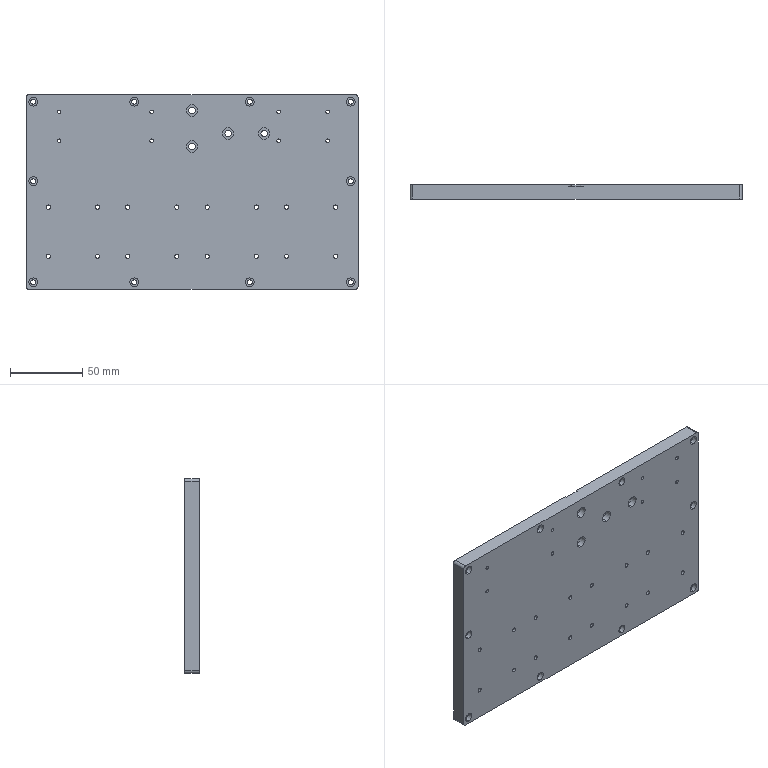CAM job | Mastercam | mm | 15 operations | part box 230 x 10 x 135
1. 2D High Speed (2D Dynamic Contour Mill) | 9 - 10C 平底刀
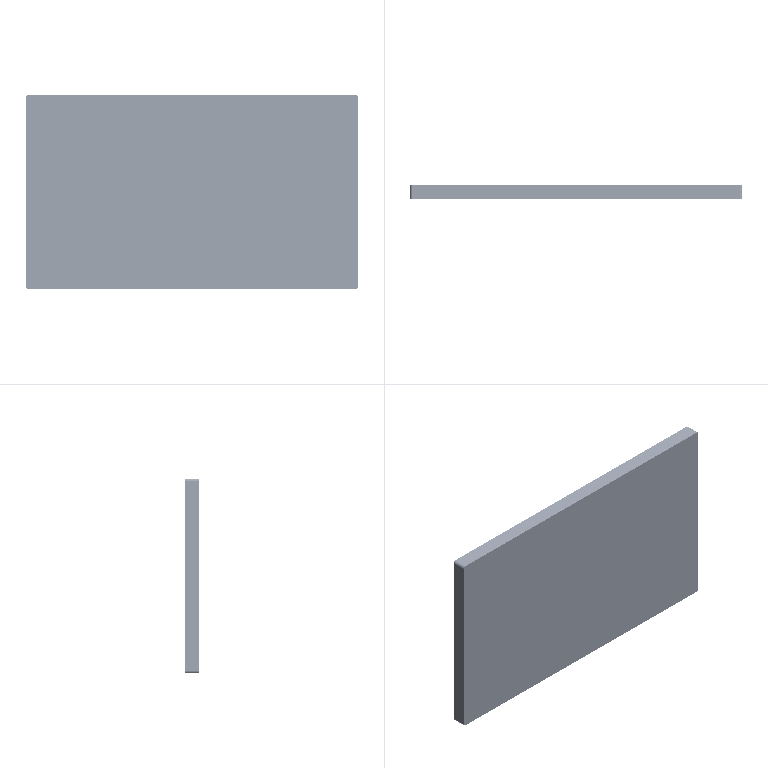2. Contour (2D) | 10 - 10J 平底刀
3. Drill/Counterbore | 2 - 6定位倒角
4. Peck Drill | 12 - 2.5 钻头
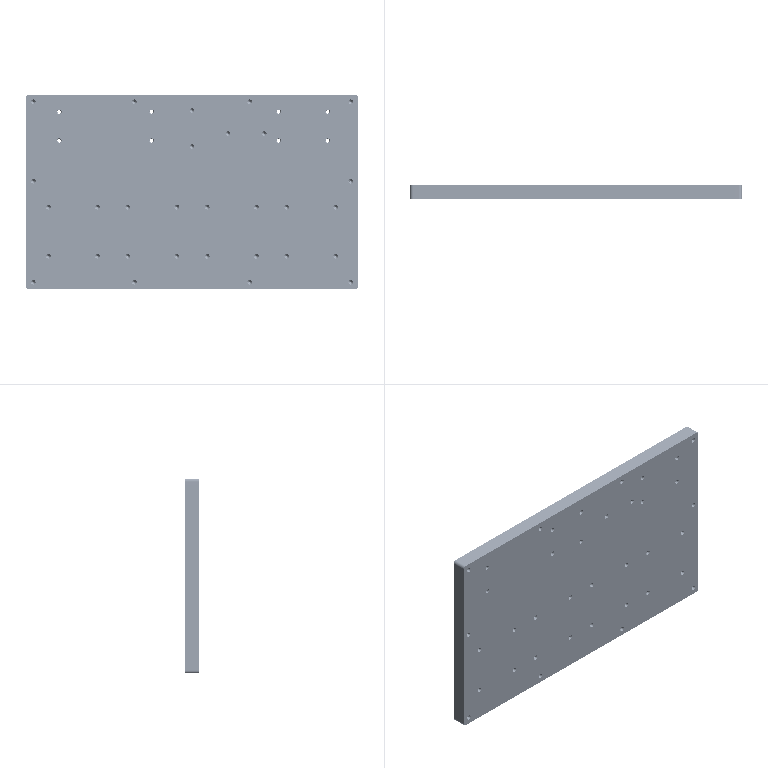5. Peck Drill | 18 - 4.5 钻头
6. Peck Drill | 13 - 3.4 钻头
7. Peck Drill | 19 - 3 钻头
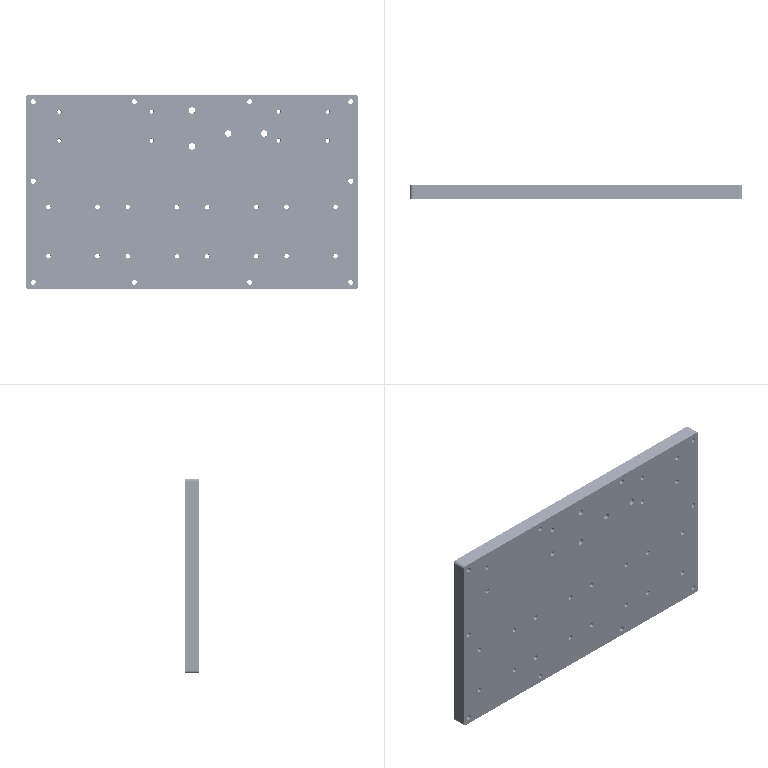8. Helix Bore | 7 - 4 平底刀
9. Model Chamfer | 2 - 6定位倒角
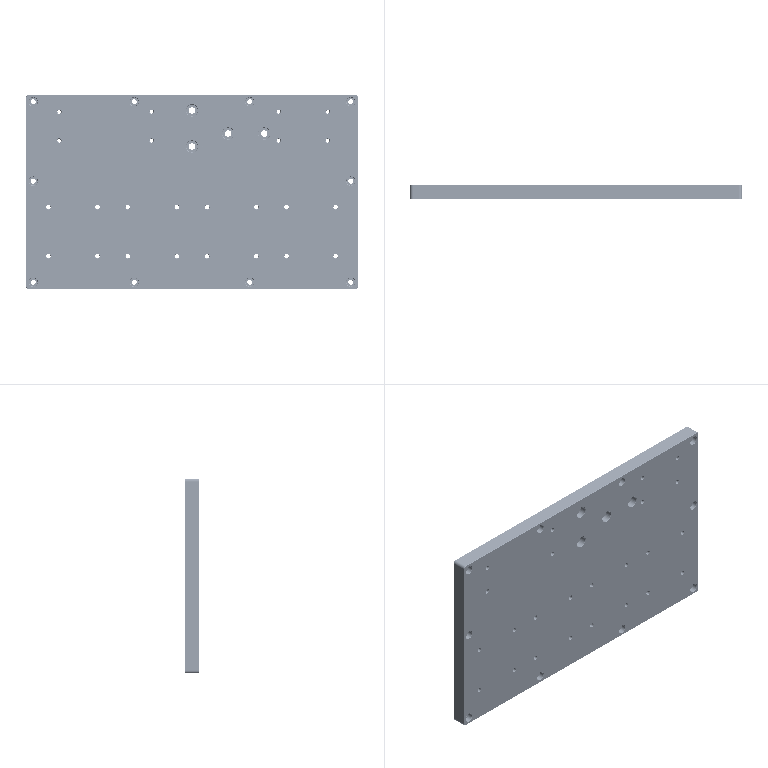10. Helix Bore | 12 - 3 平铣刀
11. Pocket (Open) | 7 - 4 平底刀
12. Contour (Remachining) | 12 - 3 平铣刀
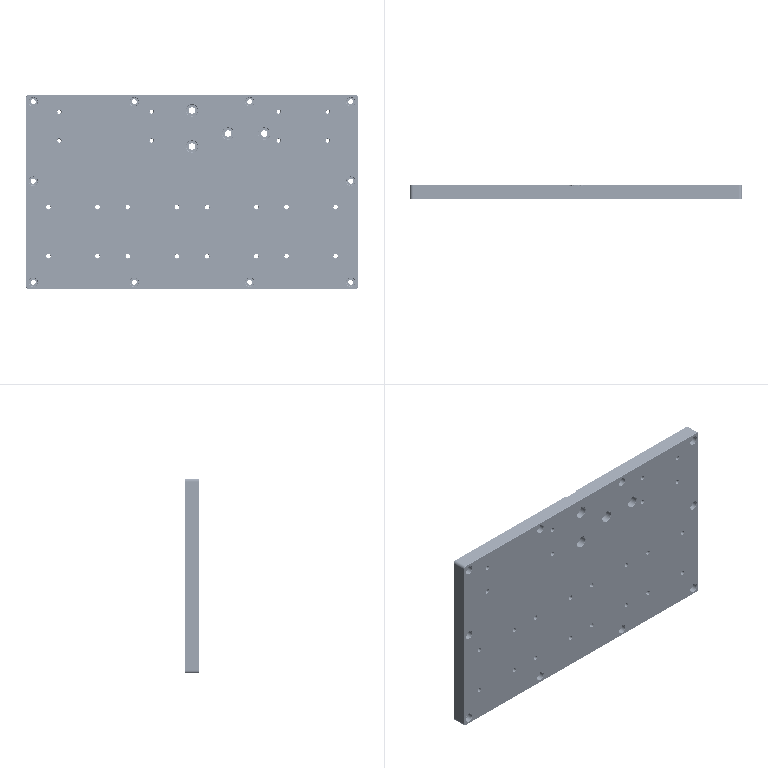13. Pocket (Open) | 12 - 3 平铣刀
14. Model Chamfer | 2 - 6定位倒角
15. Chamfer Drill | 2 - 6定位倒角